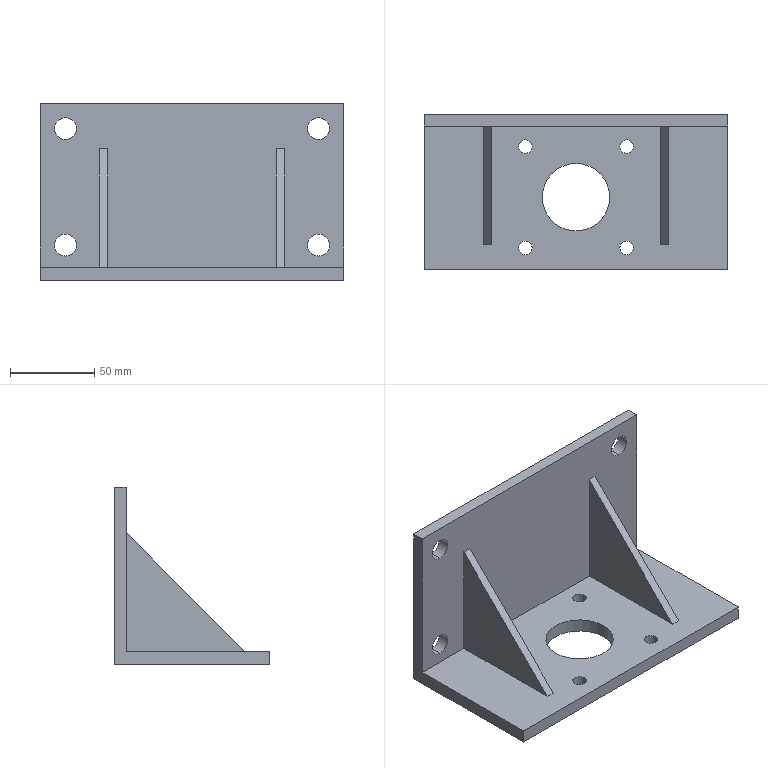Component | SolidWorks | NewTypeCurveBenderDoubleTelescopicCylinderBasePlate-DoubleWheel-2 | 1 solid | 32 faces | box 180 x 92 x 105 mm | volume 263822 mm3 | cylinder 18 | plane 14 | commonest cylinder face diameters 13 x8 8 x8 40 x2
STEP:
#1=COLOUR_RGB('',0.7922,0.8196,0.9333);
#2=FILL_AREA_STYLE_COLOUR('',#1);
#3=FILL_AREA_STYLE('',(#2));
#4=SURFACE_STYLE_FILL_AREA(#3);
#5=SURFACE_SIDE_STYLE('',(#4));
#6=SURFACE_STYLE_USAGE(.BOTH.,#5);
#7=PRESENTATION_STYLE_ASSIGNMENT((#6));
#8=CARTESIAN_POINT('',(2.953,3.504,14.04));
#9=VERTEX_POINT('',#8);
#10=CARTESIAN_POINT('',(2.953,3.504,14.552));
#11=VERTEX_POINT('',#10);
#12=CARTESIAN_POINT('',(2.953,3.504,14.296));
#13=DIRECTION('',(-0.,1.,0.));
#14=DIRECTION('',(0.,0.,1.));
#15=AXIS2_PLACEMENT_3D('',#12,#13,#14);
#16=CIRCLE('',#15,0.2559);
#17=EDGE_CURVE('',#9,#11,#16,.T.);
#18=ORIENTED_EDGE('',*,*,#17,.F.);
#19=CARTESIAN_POINT('',(2.953,3.78,14.04));
#20=VERTEX_POINT('',#19);
#21=CARTESIAN_POINT('',(2.953,3.78,14.04));
#22=DIRECTION('',(-0.,1.,0.));
#23=VECTOR('',#22,39.37);
#24=LINE('',#21,#23);
#25=EDGE_CURVE('',#9,#20,#24,.T.);
#26=ORIENTED_EDGE('',*,*,#25,.T.);
#27=CARTESIAN_POINT('',(2.953,3.78,14.552));
#28=VERTEX_POINT('',#27);
#29=CARTESIAN_POINT('',(2.953,3.78,14.296));
#30=DIRECTION('',(-0.,1.,0.));
#31=DIRECTION('',(0.,0.,1.));
#32=AXIS2_PLACEMENT_3D('',#29,#30,#31);
#33=CIRCLE('',#32,0.2559);
#34=EDGE_CURVE('',#20,#28,#33,.T.);
#35=ORIENTED_EDGE('',*,*,#34,.T.);
#36=CARTESIAN_POINT('',(2.953,3.78,14.552));
#37=DIRECTION('',(-0.,1.,0.));
#38=VECTOR('',#37,39.37);
#39=LINE('',#36,#38);
#40=EDGE_CURVE('',#11,#28,#39,.T.);
#41=ORIENTED_EDGE('',*,*,#40,.F.);
#42=EDGE_LOOP('',(#18,#26,#35,#41));
#43=FACE_OUTER_BOUND('',#42,.T.);
#44=CARTESIAN_POINT('',(2.953,3.78,14.296));
#45=DIRECTION('',(-0.,1.,0.));
#46=DIRECTION('',(0.,0.,1.));
#47=AXIS2_PLACEMENT_3D('',#44,#45,#46);
#48=CYLINDRICAL_SURFACE('',#47,0.2559);
#49=ADVANCED_FACE('',(#43),#48,.F.);
#50=CARTESIAN_POINT('',(2.953,3.504,11.323));
#51=VERTEX_POINT('',#50);
#52=CARTESIAN_POINT('',(2.953,3.504,11.835));
#53=VERTEX_POINT('',#52);
#54=CARTESIAN_POINT('',(2.953,3.504,11.579));
#55=DIRECTION('',(-0.,1.,0.));
#56=DIRECTION('',(0.,0.,1.));
#57=AXIS2_PLACEMENT_3D('',#54,#55,#56);
#58=CIRCLE('',#57,0.2559);
#59=EDGE_CURVE('',#51,#53,#58,.T.);
#60=ORIENTED_EDGE('',*,*,#59,.F.);
#61=CARTESIAN_POINT('',(2.953,3.78,11.323));
#62=VERTEX_POINT('',#61);
#63=CARTESIAN_POINT('',(2.953,3.78,11.323));
#64=DIRECTION('',(-0.,1.,0.));
#65=VECTOR('',#64,39.37);
#66=LINE('',#63,#65);
#67=EDGE_CURVE('',#51,#62,#66,.T.);
#68=ORIENTED_EDGE('',*,*,#67,.T.);
#69=CARTESIAN_POINT('',(2.953,3.78,11.835));
#70=VERTEX_POINT('',#69);
#71=CARTESIAN_POINT('',(2.953,3.78,11.579));
#72=DIRECTION('',(-0.,1.,0.));
#73=DIRECTION('',(0.,0.,1.));
#74=AXIS2_PLACEMENT_3D('',#71,#72,#73);
#75=CIRCLE('',#74,0.2559);
#76=EDGE_CURVE('',#62,#70,#75,.T.);
#77=ORIENTED_EDGE('',*,*,#76,.T.);
#78=CARTESIAN_POINT('',(2.953,3.78,11.835));
#79=DIRECTION('',(-0.,1.,0.));
#80=VECTOR('',#79,39.37);
#81=LINE('',#78,#80);
#82=EDGE_CURVE('',#53,#70,#81,.T.);
#83=ORIENTED_EDGE('',*,*,#82,.F.);
#84=EDGE_LOOP('',(#60,#68,#77,#83));
#85=FACE_OUTER_BOUND('',#84,.T.);
#86=CARTESIAN_POINT('',(2.953,3.78,11.579));
#87=DIRECTION('',(-0.,1.,0.));
#88=DIRECTION('',(0.,0.,1.));
#89=AXIS2_PLACEMENT_3D('',#86,#87,#88);
#90=CYLINDRICAL_SURFACE('',#89,0.2559);
#91=ADVANCED_FACE('',(#85),#90,.F.);
#92=CARTESIAN_POINT('',(-2.953,3.504,11.323));
#93=VERTEX_POINT('',#92);
#94=CARTESIAN_POINT('',(-2.953,3.504,11.835));
#95=VERTEX_POINT('',#94);
#96=CARTESIAN_POINT('',(-2.953,3.504,11.579));
#97=DIRECTION('',(-0.,1.,0.));
#98=DIRECTION('',(0.,0.,1.));
#99=AXIS2_PLACEMENT_3D('',#96,#97,#98);
#100=CIRCLE('',#99,0.2559);
#101=EDGE_CURVE('',#93,#95,#100,.T.);
#102=ORIENTED_EDGE('',*,*,#101,.F.);
#103=CARTESIAN_POINT('',(-2.953,3.78,11.323));
#104=VERTEX_POINT('',#103);
#105=CARTESIAN_POINT('',(-2.953,3.78,11.323));
#106=DIRECTION('',(-0.,1.,0.));
#107=VECTOR('',#106,39.37);
#108=LINE('',#105,#107);
#109=EDGE_CURVE('',#93,#104,#108,.T.);
#110=ORIENTED_EDGE('',*,*,#109,.T.);
#111=CARTESIAN_POINT('',(-2.953,3.78,11.835));
#112=VERTEX_POINT('',#111);
#113=CARTESIAN_POINT('',(-2.953,3.78,11.579));
#114=DIRECTION('',(-0.,1.,0.));
#115=DIRECTION('',(0.,0.,1.));
#116=AXIS2_PLACEMENT_3D('',#113,#114,#115);
#117=CIRCLE('',#116,0.2559);
#118=EDGE_CURVE('',#104,#112,#117,.T.);
#119=ORIENTED_EDGE('',*,*,#118,.T.);
#120=CARTESIAN_POINT('',(-2.953,3.78,11.835));
#121=DIRECTION('',(-0.,1.,0.));
#122=VECTOR('',#121,39.37);
#123=LINE('',#120,#122);
#124=EDGE_CURVE('',#95,#112,#123,.T.);
#125=ORIENTED_EDGE('',*,*,#124,.F.);
#126=EDGE_LOOP('',(#102,#110,#119,#125));
#127=FACE_OUTER_BOUND('',#126,.T.);
#128=CARTESIAN_POINT('',(-2.953,3.78,11.579));
#129=DIRECTION('',(-0.,1.,0.));
#130=DIRECTION('',(0.,0.,1.));
#131=AXIS2_PLACEMENT_3D('',#128,#129,#130);
#132=CYLINDRICAL_SURFACE('',#131,0.2559);
#133=ADVANCED_FACE('',(#127),#132,.F.);
#134=CARTESIAN_POINT('',(-2.953,3.504,14.04));
#135=VERTEX_POINT('',#134);
#136=CARTESIAN_POINT('',(-2.953,3.504,14.552));
#137=VERTEX_POINT('',#136);
#138=CARTESIAN_POINT('',(-2.953,3.504,14.296));
#139=DIRECTION('',(-0.,1.,0.));
#140=DIRECTION('',(0.,0.,1.));
#141=AXIS2_PLACEMENT_3D('',#138,#139,#140);
#142=CIRCLE('',#141,0.2559);
#143=EDGE_CURVE('',#135,#137,#142,.T.);
#144=ORIENTED_EDGE('',*,*,#143,.F.);
#145=CARTESIAN_POINT('',(-2.953,3.78,14.04));
#146=VERTEX_POINT('',#145);
#147=CARTESIAN_POINT('',(-2.953,3.78,14.04));
#148=DIRECTION('',(-0.,1.,0.));
#149=VECTOR('',#148,39.37);
#150=LINE('',#147,#149);
#151=EDGE_CURVE('',#135,#146,#150,.T.);
#152=ORIENTED_EDGE('',*,*,#151,.T.);
#153=CARTESIAN_POINT('',(-2.953,3.78,14.552));
#154=VERTEX_POINT('',#153);
#155=CARTESIAN_POINT('',(-2.953,3.78,14.296));
#156=DIRECTION('',(-0.,1.,0.));
#157=DIRECTION('',(0.,0.,1.));
#158=AXIS2_PLACEMENT_3D('',#155,#156,#157);
#159=CIRCLE('',#158,0.2559);
#160=EDGE_CURVE('',#146,#154,#159,.T.);
#161=ORIENTED_EDGE('',*,*,#160,.T.);
#162=CARTESIAN_POINT('',(-2.953,3.78,14.552));
#163=DIRECTION('',(-0.,1.,0.));
#164=VECTOR('',#163,39.37);
#165=LINE('',#162,#164);
#166=EDGE_CURVE('',#137,#154,#165,.T.);
#167=ORIENTED_EDGE('',*,*,#166,.F.);
#168=EDGE_LOOP('',(#144,#152,#161,#167));
#169=FACE_OUTER_BOUND('',#168,.T.);
#170=CARTESIAN_POINT('',(-2.953,3.78,14.296));
#171=DIRECTION('',(-0.,1.,0.));
#172=DIRECTION('',(0.,0.,1.));
#173=AXIS2_PLACEMENT_3D('',#170,#171,#172);
#174=CYLINDRICAL_SURFACE('',#173,0.2559);
#175=ADVANCED_FACE('',(#169),#174,.F.);
#176=CARTESIAN_POINT('',(-1.339,3.031,11.067));
#177=VERTEX_POINT('',#176);
#178=CARTESIAN_POINT('',(-1.024,3.031,11.067));
#179=VERTEX_POINT('',#178);
#180=CARTESIAN_POINT('',(-1.181,3.031,11.067));
#181=DIRECTION('',(-0.,0.,-1.));
#182=DIRECTION('',(1.,0.,0.));
#183=AXIS2_PLACEMENT_3D('',#180,#181,#182);
#184=CIRCLE('',#183,0.1575);
#185=EDGE_CURVE('',#177,#179,#184,.T.);
#186=ORIENTED_EDGE('',*,*,#185,.F.);
#187=CARTESIAN_POINT('',(-1.339,3.031,10.752));
#188=VERTEX_POINT('',#187);
#189=CARTESIAN_POINT('',(-1.339,3.031,11.146));
#190=DIRECTION('',(-0.,0.,-1.));
#191=VECTOR('',#190,39.37);
#192=LINE('',#189,#191);
#193=EDGE_CURVE('',#177,#188,#192,.T.);
#194=ORIENTED_EDGE('',*,*,#193,.T.);
#195=CARTESIAN_POINT('',(-1.024,3.031,10.752));
#196=VERTEX_POINT('',#195);
#197=CARTESIAN_POINT('',(-1.181,3.031,10.752));
#198=DIRECTION('',(-0.,0.,-1.));
#199=DIRECTION('',(-1.,0.,0.));
#200=AXIS2_PLACEMENT_3D('',#197,#198,#199);
#201=CIRCLE('',#200,0.1575);
#202=EDGE_CURVE('',#188,#196,#201,.T.);
#203=ORIENTED_EDGE('',*,*,#202,.T.);
#204=CARTESIAN_POINT('',(-1.024,3.031,11.146));
#205=DIRECTION('',(-0.,0.,-1.));
#206=VECTOR('',#205,39.37);
#207=LINE('',#204,#206);
#208=EDGE_CURVE('',#179,#196,#207,.T.);
#209=ORIENTED_EDGE('',*,*,#208,.F.);
#210=EDGE_LOOP('',(#186,#194,#203,#209));
#211=FACE_OUTER_BOUND('',#210,.T.);
#212=CARTESIAN_POINT('',(-1.181,3.031,11.146));
#213=DIRECTION('',(-0.,0.,-1.));
#214=DIRECTION('',(1.,0.,0.));
#215=AXIS2_PLACEMENT_3D('',#212,#213,#214);
#216=CYLINDRICAL_SURFACE('',#215,0.1575);
#217=ADVANCED_FACE('',(#211),#216,.F.);
#218=CARTESIAN_POINT('',(1.024,3.031,11.067));
#219=VERTEX_POINT('',#218);
#220=CARTESIAN_POINT('',(1.339,3.031,11.067));
#221=VERTEX_POINT('',#220);
#222=CARTESIAN_POINT('',(1.181,3.031,11.067));
#223=DIRECTION('',(-0.,0.,-1.));
#224=DIRECTION('',(1.,0.,0.));
#225=AXIS2_PLACEMENT_3D('',#222,#223,#224);
#226=CIRCLE('',#225,0.1575);
#227=EDGE_CURVE('',#219,#221,#226,.T.);
#228=ORIENTED_EDGE('',*,*,#227,.F.);
#229=CARTESIAN_POINT('',(1.024,3.031,10.752));
#230=VERTEX_POINT('',#229);
#231=CARTESIAN_POINT('',(1.024,3.031,11.146));
#232=DIRECTION('',(-0.,0.,-1.));
#233=VECTOR('',#232,39.37);
#234=LINE('',#231,#233);
#235=EDGE_CURVE('',#219,#230,#234,.T.);
#236=ORIENTED_EDGE('',*,*,#235,.T.);
#237=CARTESIAN_POINT('',(1.339,3.031,10.752));
#238=VERTEX_POINT('',#237);
#239=CARTESIAN_POINT('',(1.181,3.031,10.752));
#240=DIRECTION('',(-0.,0.,-1.));
#241=DIRECTION('',(1.,0.,0.));
#242=AXIS2_PLACEMENT_3D('',#239,#240,#241);
#243=CIRCLE('',#242,0.1575);
#244=EDGE_CURVE('',#230,#238,#243,.T.);
#245=ORIENTED_EDGE('',*,*,#244,.T.);
#246=CARTESIAN_POINT('',(1.339,3.031,11.146));
#247=DIRECTION('',(-0.,0.,-1.));
#248=VECTOR('',#247,39.37);
#249=LINE('',#246,#248);
#250=EDGE_CURVE('',#221,#238,#249,.T.);
#251=ORIENTED_EDGE('',*,*,#250,.F.);
#252=EDGE_LOOP('',(#228,#236,#245,#251));
#253=FACE_OUTER_BOUND('',#252,.T.);
#254=CARTESIAN_POINT('',(1.181,3.031,11.146));
#255=DIRECTION('',(-0.,0.,-1.));
#256=DIRECTION('',(1.,0.,0.));
#257=AXIS2_PLACEMENT_3D('',#254,#255,#256);
#258=CYLINDRICAL_SURFACE('',#257,0.1575);
#259=ADVANCED_FACE('',(#253),#258,.F.);
#260=CARTESIAN_POINT('',(1.024,0.6693,11.067));
#261=VERTEX_POINT('',#260);
#262=CARTESIAN_POINT('',(1.339,0.6693,11.067));
#263=VERTEX_POINT('',#262);
#264=CARTESIAN_POINT('',(1.181,0.6693,11.067));
#265=DIRECTION('',(-0.,0.,-1.));
#266=DIRECTION('',(1.,0.,0.));
#267=AXIS2_PLACEMENT_3D('',#264,#265,#266);
#268=CIRCLE('',#267,0.1575);
#269=EDGE_CURVE('',#261,#263,#268,.T.);
#270=ORIENTED_EDGE('',*,*,#269,.F.);
#271=CARTESIAN_POINT('',(1.024,0.6693,10.752));
#272=VERTEX_POINT('',#271);
#273=CARTESIAN_POINT('',(1.024,0.6693,11.146));
#274=DIRECTION('',(-0.,0.,-1.));
#275=VECTOR('',#274,39.37);
#276=LINE('',#273,#275);
#277=EDGE_CURVE('',#261,#272,#276,.T.);
#278=ORIENTED_EDGE('',*,*,#277,.T.);
#279=CARTESIAN_POINT('',(1.339,0.6693,10.752));
#280=VERTEX_POINT('',#279);
#281=CARTESIAN_POINT('',(1.181,0.6693,10.752));
#282=DIRECTION('',(-0.,0.,-1.));
#283=DIRECTION('',(-1.,0.,0.));
#284=AXIS2_PLACEMENT_3D('',#281,#282,#283);
#285=CIRCLE('',#284,0.1575);
#286=EDGE_CURVE('',#272,#280,#285,.T.);
#287=ORIENTED_EDGE('',*,*,#286,.T.);
#288=CARTESIAN_POINT('',(1.339,0.6693,11.146));
#289=DIRECTION('',(-0.,0.,-1.));
#290=VECTOR('',#289,39.37);
#291=LINE('',#288,#290);
#292=EDGE_CURVE('',#263,#280,#291,.T.);
#293=ORIENTED_EDGE('',*,*,#292,.F.);
#294=EDGE_LOOP('',(#270,#278,#287,#293));
#295=FACE_OUTER_BOUND('',#294,.T.);
#296=CARTESIAN_POINT('',(1.181,0.6693,11.146));
#297=DIRECTION('',(-0.,0.,-1.));
#298=DIRECTION('',(1.,0.,0.));
#299=AXIS2_PLACEMENT_3D('',#296,#297,#298);
#300=CYLINDRICAL_SURFACE('',#299,0.1575);
#301=ADVANCED_FACE('',(#295),#300,.F.);
#302=CARTESIAN_POINT('',(-1.339,0.6693,11.067));
#303=VERTEX_POINT('',#302);
#304=CARTESIAN_POINT('',(-1.024,0.6693,11.067));
#305=VERTEX_POINT('',#304);
#306=CARTESIAN_POINT('',(-1.181,0.6693,11.067));
#307=DIRECTION('',(-0.,0.,-1.));
#308=DIRECTION('',(1.,0.,0.));
#309=AXIS2_PLACEMENT_3D('',#306,#307,#308);
#310=CIRCLE('',#309,0.1575);
#311=EDGE_CURVE('',#303,#305,#310,.T.);
#312=ORIENTED_EDGE('',*,*,#311,.F.);
#313=CARTESIAN_POINT('',(-1.339,0.6693,10.752));
#314=VERTEX_POINT('',#313);
#315=CARTESIAN_POINT('',(-1.339,0.6693,11.146));
#316=DIRECTION('',(-0.,0.,-1.));
#317=VECTOR('',#316,39.37);
#318=LINE('',#315,#317);
#319=EDGE_CURVE('',#303,#314,#318,.T.);
#320=ORIENTED_EDGE('',*,*,#319,.T.);
#321=CARTESIAN_POINT('',(-1.024,0.6693,10.752));
#322=VERTEX_POINT('',#321);
#323=CARTESIAN_POINT('',(-1.181,0.6693,10.752));
#324=DIRECTION('',(-0.,0.,-1.));
#325=DIRECTION('',(1.,0.,0.));
#326=AXIS2_PLACEMENT_3D('',#323,#324,#325);
#327=CIRCLE('',#326,0.1575);
#328=EDGE_CURVE('',#314,#322,#327,.T.);
#329=ORIENTED_EDGE('',*,*,#328,.T.);
#330=CARTESIAN_POINT('',(-1.024,0.6693,11.146));
#331=DIRECTION('',(-0.,0.,-1.));
#332=VECTOR('',#331,39.37);
#333=LINE('',#330,#332);
#334=EDGE_CURVE('',#305,#322,#333,.T.);
#335=ORIENTED_EDGE('',*,*,#334,.F.);
#336=EDGE_LOOP('',(#312,#320,#329,#335));
#337=FACE_OUTER_BOUND('',#336,.T.);
#338=CARTESIAN_POINT('',(-1.181,0.6693,11.146));
#339=DIRECTION('',(-0.,0.,-1.));
#340=DIRECTION('',(1.,0.,0.));
#341=AXIS2_PLACEMENT_3D('',#338,#339,#340);
#342=CYLINDRICAL_SURFACE('',#341,0.1575);
#343=ADVANCED_FACE('',(#337),#342,.F.);
#344=CARTESIAN_POINT('',(-0.7874,1.85,11.067));
#345=VERTEX_POINT('',#344);
#346=CARTESIAN_POINT('',(0.7874,1.85,11.067));
#347=VERTEX_POINT('',#346);
#348=CARTESIAN_POINT('',(-0.,1.85,11.067));
#349=DIRECTION('',(-0.,0.,-1.));
#350=DIRECTION('',(1.,0.,0.));
#351=AXIS2_PLACEMENT_3D('',#348,#349,#350);
#352=CIRCLE('',#351,0.7874);
#353=EDGE_CURVE('',#345,#347,#352,.T.);
#354=ORIENTED_EDGE('',*,*,#353,.F.);
#355=CARTESIAN_POINT('',(-0.7874,1.85,10.752));
#356=VERTEX_POINT('',#355);
#357=CARTESIAN_POINT('',(-0.7874,1.85,11.146));
#358=DIRECTION('',(-0.,0.,-1.));
#359=VECTOR('',#358,39.37);
#360=LINE('',#357,#359);
#361=EDGE_CURVE('',#345,#356,#360,.T.);
#362=ORIENTED_EDGE('',*,*,#361,.T.);
#363=CARTESIAN_POINT('',(0.7874,1.85,10.752));
#364=VERTEX_POINT('',#363);
#365=CARTESIAN_POINT('',(-0.,1.85,10.752));
#366=DIRECTION('',(-0.,0.,-1.));
#367=DIRECTION('',(1.,0.,0.));
#368=AXIS2_PLACEMENT_3D('',#365,#366,#367);
#369=CIRCLE('',#368,0.7874);
#370=EDGE_CURVE('',#356,#364,#369,.T.);
#371=ORIENTED_EDGE('',*,*,#370,.T.);
#372=CARTESIAN_POINT('',(0.7874,1.85,11.146));
#373=DIRECTION('',(-0.,0.,-1.));
#374=VECTOR('',#373,39.37);
#375=LINE('',#372,#374);
#376=EDGE_CURVE('',#347,#364,#375,.T.);
#377=ORIENTED_EDGE('',*,*,#376,.F.);
#378=EDGE_LOOP('',(#354,#362,#371,#377));
#379=FACE_OUTER_BOUND('',#378,.T.);
#380=CARTESIAN_POINT('',(-0.,1.85,11.146));
#381=DIRECTION('',(-0.,0.,-1.));
#382=DIRECTION('',(1.,0.,0.));
#383=AXIS2_PLACEMENT_3D('',#380,#381,#382);
#384=CYLINDRICAL_SURFACE('',#383,0.7874);
#385=ADVANCED_FACE('',(#379),#384,.F.);
#386=CARTESIAN_POINT('',(-0.,1.85,11.067));
#387=DIRECTION('',(-0.,0.,-1.));
#388=DIRECTION('',(1.,0.,0.));
#389=AXIS2_PLACEMENT_3D('',#386,#387,#388);
#390=CIRCLE('',#389,0.7874);
#391=EDGE_CURVE('',#347,#345,#390,.T.);
#392=ORIENTED_EDGE('',*,*,#391,.T.);
#393=ORIENTED_EDGE('',*,*,#353,.T.);
#394=EDGE_LOOP('',(#392,#393));
#395=FACE_BOUND('',#394,.T.);
#396=CARTESIAN_POINT('',(-1.181,0.6693,11.067));
#397=DIRECTION('',(-0.,0.,-1.));
#398=DIRECTION('',(1.,0.,0.));
#399=AXIS2_PLACEMENT_3D('',#396,#397,#398);
#400=CIRCLE('',#399,0.1575);
#401=EDGE_CURVE('',#305,#303,#400,.T.);
#402=ORIENTED_EDGE('',*,*,#401,.T.);
#403=ORIENTED_EDGE('',*,*,#311,.T.);
#404=EDGE_LOOP('',(#402,#403));
#405=FACE_BOUND('',#404,.T.);
#406=CARTESIAN_POINT('',(1.181,0.6693,11.067));
#407=DIRECTION('',(-0.,0.,-1.));
#408=DIRECTION('',(1.,0.,0.));
#409=AXIS2_PLACEMENT_3D('',#406,#407,#408);
#410=CIRCLE('',#409,0.1575);
#411=EDGE_CURVE('',#263,#261,#410,.T.);
#412=ORIENTED_EDGE('',*,*,#411,.T.);
#413=ORIENTED_EDGE('',*,*,#269,.T.);
#414=EDGE_LOOP('',(#412,#413));
#415=FACE_BOUND('',#414,.T.);
#416=CARTESIAN_POINT('',(1.181,3.031,11.067));
#417=DIRECTION('',(-0.,0.,-1.));
#418=DIRECTION('',(1.,0.,0.));
#419=AXIS2_PLACEMENT_3D('',#416,#417,#418);
#420=CIRCLE('',#419,0.1575);
#421=EDGE_CURVE('',#221,#219,#420,.T.);
#422=ORIENTED_EDGE('',*,*,#421,.T.);
#423=ORIENTED_EDGE('',*,*,#227,.T.);
#424=EDGE_LOOP('',(#422,#423));
#425=FACE_BOUND('',#424,.T.);
#426=CARTESIAN_POINT('',(-1.181,3.031,11.067));
#427=DIRECTION('',(-0.,0.,-1.));
#428=DIRECTION('',(1.,0.,0.));
#429=AXIS2_PLACEMENT_3D('',#426,#427,#428);
#430=CIRCLE('',#429,0.1575);
#431=EDGE_CURVE('',#179,#177,#430,.T.);
#432=ORIENTED_EDGE('',*,*,#431,.T.);
#433=ORIENTED_EDGE('',*,*,#185,.T.);
#434=EDGE_LOOP('',(#432,#433));
#435=FACE_BOUND('',#434,.T.);
#436=CARTESIAN_POINT('',(1.969,0.748,11.067));
#437=VERTEX_POINT('',#436);
#438=CARTESIAN_POINT('',(2.165,0.748,11.067));
#439=VERTEX_POINT('',#438);
#440=CARTESIAN_POINT('',(1.969,0.748,11.067));
#441=DIRECTION('',(1.,0.,-0.));
#442=VECTOR('',#441,39.37);
#443=LINE('',#440,#442);
#444=EDGE_CURVE('',#437,#439,#443,.T.);
#445=ORIENTED_EDGE('',*,*,#444,.F.);
#446=CARTESIAN_POINT('',(1.969,3.504,11.067));
#447=VERTEX_POINT('',#446);
#448=CARTESIAN_POINT('',(1.969,3.504,11.067));
#449=DIRECTION('',(0.,-1.,-0.));
#450=VECTOR('',#449,39.37);
#451=LINE('',#448,#450);
#452=EDGE_CURVE('',#447,#437,#451,.T.);
#453=ORIENTED_EDGE('',*,*,#452,.F.);
#454=CARTESIAN_POINT('',(-1.969,3.504,11.067));
#455=VERTEX_POINT('',#454);
#456=CARTESIAN_POINT('',(3.543,3.504,11.067));
#457=DIRECTION('',(1.,0.,-0.));
#458=VECTOR('',#457,39.37);
#459=LINE('',#456,#458);
#460=EDGE_CURVE('',#455,#447,#459,.T.);
#461=ORIENTED_EDGE('',*,*,#460,.F.);
#462=CARTESIAN_POINT('',(-1.969,0.748,11.067));
#463=VERTEX_POINT('',#462);
#464=CARTESIAN_POINT('',(-1.969,3.504,11.067));
#465=DIRECTION('',(-0.,-1.,-0.));
#466=VECTOR('',#465,39.37);
#467=LINE('',#464,#466);
#468=EDGE_CURVE('',#455,#463,#467,.T.);
#469=ORIENTED_EDGE('',*,*,#468,.T.);
#470=CARTESIAN_POINT('',(-2.165,0.748,11.067));
#471=VERTEX_POINT('',#470);
#472=CARTESIAN_POINT('',(-1.969,0.748,11.067));
#473=DIRECTION('',(-1.,0.,0.));
#474=VECTOR('',#473,39.37);
#475=LINE('',#472,#474);
#476=EDGE_CURVE('',#463,#471,#475,.T.);
#477=ORIENTED_EDGE('',*,*,#476,.T.);
#478=CARTESIAN_POINT('',(-2.165,3.504,11.067));
#479=VERTEX_POINT('',#478);
#480=CARTESIAN_POINT('',(-2.165,3.504,11.067));
#481=DIRECTION('',(-0.,-1.,-0.));
#482=VECTOR('',#481,39.37);
#483=LINE('',#480,#482);
#484=EDGE_CURVE('',#479,#471,#483,.T.);
#485=ORIENTED_EDGE('',*,*,#484,.F.);
#486=CARTESIAN_POINT('',(-3.543,3.504,11.067));
#487=VERTEX_POINT('',#486);
#488=CARTESIAN_POINT('',(3.543,3.504,11.067));
#489=DIRECTION('',(1.,0.,-0.));
#490=VECTOR('',#489,39.37);
#491=LINE('',#488,#490);
#492=EDGE_CURVE('',#487,#479,#491,.T.);
#493=ORIENTED_EDGE('',*,*,#492,.F.);
#494=CARTESIAN_POINT('',(-3.543,0.1575,11.067));
#495=VERTEX_POINT('',#494);
#496=CARTESIAN_POINT('',(-3.543,0.1575,11.067));
#497=DIRECTION('',(-0.,1.,0.));
#498=VECTOR('',#497,39.37);
#499=LINE('',#496,#498);
#500=EDGE_CURVE('',#495,#487,#499,.T.);
#501=ORIENTED_EDGE('',*,*,#500,.F.);
#502=CARTESIAN_POINT('',(3.543,0.1575,11.067));
#503=VERTEX_POINT('',#502);
#504=CARTESIAN_POINT('',(-3.543,0.1575,11.067));
#505=DIRECTION('',(-1.,-0.,0.));
#506=VECTOR('',#505,39.37);
#507=LINE('',#504,#506);
#508=EDGE_CURVE('',#503,#495,#507,.T.);
#509=ORIENTED_EDGE('',*,*,#508,.F.);
#510=CARTESIAN_POINT('',(3.543,3.504,11.067));
#511=VERTEX_POINT('',#510);
#512=CARTESIAN_POINT('',(3.543,0.1575,11.067));
#513=DIRECTION('',(0.,-1.,-0.));
#514=VECTOR('',#513,39.37);
#515=LINE('',#512,#514);
#516=EDGE_CURVE('',#511,#503,#515,.T.);
#517=ORIENTED_EDGE('',*,*,#516,.F.);
#518=CARTESIAN_POINT('',(2.165,3.504,11.067));
#519=VERTEX_POINT('',#518);
#520=CARTESIAN_POINT('',(3.543,3.504,11.067));
#521=DIRECTION('',(1.,0.,-0.));
#522=VECTOR('',#521,39.37);
#523=LINE('',#520,#522);
#524=EDGE_CURVE('',#519,#511,#523,.T.);
#525=ORIENTED_EDGE('',*,*,#524,.F.);
#526=CARTESIAN_POINT('',(2.165,3.504,11.067));
#527=DIRECTION('',(0.,-1.,-0.));
#528=VECTOR('',#527,39.37);
#529=LINE('',#526,#528);
#530=EDGE_CURVE('',#519,#439,#529,.T.);
#531=ORIENTED_EDGE('',*,*,#530,.T.);
#532=EDGE_LOOP('',(#445,#453,#461,#469,#477,#485,#493,#501,#509,#517,#525,#531));
#533=FACE_OUTER_BOUND('',#532,.T.);
#534=CARTESIAN_POINT('',(-0.,1.988,11.067));
#535=DIRECTION('',(-0.,0.,-1.));
#536=DIRECTION('',(1.,0.,-0.));
#537=AXIS2_PLACEMENT_3D('',#534,#535,#536);
#538=PLANE('',#537);
#539=ADVANCED_FACE('',(#395,#405,#415,#425,#435,#533),#538,.F.);
#540=CARTESIAN_POINT('',(3.543,3.78,10.752));
#541=VERTEX_POINT('',#540);
#542=CARTESIAN_POINT('',(3.543,0.1575,10.752));
#543=VERTEX_POINT('',#542);
#544=CARTESIAN_POINT('',(3.543,0.1575,10.752));
#545=DIRECTION('',(0.,-1.,-0.));
#546=VECTOR('',#545,39.37);
#547=LINE('',#544,#546);
#548=EDGE_CURVE('',#541,#543,#547,.T.);
#549=ORIENTED_EDGE('',*,*,#548,.F.);
#550=CARTESIAN_POINT('',(3.543,3.78,14.886));
#551=VERTEX_POINT('',#550);
#552=CARTESIAN_POINT('',(3.543,3.78,14.886));
#553=DIRECTION('',(-0.,0.,-1.));
#554=VECTOR('',#553,39.37);
#555=LINE('',#552,#554);
#556=EDGE_CURVE('',#551,#541,#555,.T.);
#557=ORIENTED_EDGE('',*,*,#556,.F.);
#558=CARTESIAN_POINT('',(3.543,3.504,14.886));
#559=VERTEX_POINT('',#558);
#560=CARTESIAN_POINT('',(3.543,3.78,14.886));
#561=DIRECTION('',(-0.,1.,0.));
#562=VECTOR('',#561,39.37);
#563=LINE('',#560,#562);
#564=EDGE_CURVE('',#559,#551,#563,.T.);
#565=ORIENTED_EDGE('',*,*,#564,.F.);
#566=CARTESIAN_POINT('',(3.543,3.504,14.886));
#567=DIRECTION('',(-0.,0.,-1.));
#568=VECTOR('',#567,39.37);
#569=LINE('',#566,#568);
#570=EDGE_CURVE('',#559,#511,#569,.T.);
#571=ORIENTED_EDGE('',*,*,#570,.T.);
#572=ORIENTED_EDGE('',*,*,#516,.T.);
#573=CARTESIAN_POINT('',(3.543,0.1575,10.752));
#574=DIRECTION('',(0.,-0.,1.));
#575=VECTOR('',#574,39.37);
#576=LINE('',#573,#575);
#577=EDGE_CURVE('',#543,#503,#576,.T.);
#578=ORIENTED_EDGE('',*,*,#577,.F.);
#579=EDGE_LOOP('',(#549,#557,#565,#571,#572,#578));
#580=FACE_OUTER_BOUND('',#579,.T.);
#581=CARTESIAN_POINT('',(3.543,0.1575,10.752));
#582=DIRECTION('',(-1.,-0.,0.));
#583=DIRECTION('',(-0.,0.,-1.));
#584=AXIS2_PLACEMENT_3D('',#581,#582,#583);
#585=PLANE('',#584);
#586=ADVANCED_FACE('',(#580),#585,.F.);
#587=ORIENTED_EDGE('',*,*,#508,.T.);
#588=CARTESIAN_POINT('',(-3.543,0.1575,10.752));
#589=VERTEX_POINT('',#588);
#590=CARTESIAN_POINT('',(-3.543,0.1575,10.752));
#591=DIRECTION('',(0.,-0.,1.));
#592=VECTOR('',#591,39.37);
#593=LINE('',#590,#592);
#594=EDGE_CURVE('',#589,#495,#593,.T.);
#595=ORIENTED_EDGE('',*,*,#594,.F.);
#596=CARTESIAN_POINT('',(-3.543,0.1575,10.752));
#597=DIRECTION('',(-1.,-0.,0.));
#598=VECTOR('',#597,39.37);
#599=LINE('',#596,#598);
#600=EDGE_CURVE('',#543,#589,#599,.T.);
#601=ORIENTED_EDGE('',*,*,#600,.F.);
#602=ORIENTED_EDGE('',*,*,#577,.T.);
#603=EDGE_LOOP('',(#587,#595,#601,#602));
#604=FACE_OUTER_BOUND('',#603,.T.);
#605=CARTESIAN_POINT('',(-3.543,0.1575,10.752));
#606=DIRECTION('',(-0.,1.,0.));
#607=DIRECTION('',(0.,-0.,1.));
#608=AXIS2_PLACEMENT_3D('',#605,#606,#607);
#609=PLANE('',#608);
#610=ADVANCED_FACE('',(#604),#609,.F.);
#611=CARTESIAN_POINT('',(-3.543,3.78,14.886));
#612=VERTEX_POINT('',#611);
#613=CARTESIAN_POINT('',(-3.543,3.78,10.752));
#614=VERTEX_POINT('',#613);
#615=CARTESIAN_POINT('',(-3.543,3.78,14.886));
#616=DIRECTION('',(-0.,0.,-1.));
#617=VECTOR('',#616,39.37);
#618=LINE('',#615,#617);
#619=EDGE_CURVE('',#612,#614,#618,.T.);
#620=ORIENTED_EDGE('',*,*,#619,.T.);
#621=CARTESIAN_POINT('',(-3.543,0.1575,10.752));
#622=DIRECTION('',(-0.,1.,0.));
#623=VECTOR('',#622,39.37);
#624=LINE('',#621,#623);
#625=EDGE_CURVE('',#589,#614,#624,.T.);
#626=ORIENTED_EDGE('',*,*,#625,.F.);
#627=ORIENTED_EDGE('',*,*,#594,.T.);
#628=ORIENTED_EDGE('',*,*,#500,.T.);
#629=CARTESIAN_POINT('',(-3.543,3.504,14.886));
#630=VERTEX_POINT('',#629);
#631=CARTESIAN_POINT('',(-3.543,3.504,14.886));
#632=DIRECTION('',(-0.,0.,-1.));
#633=VECTOR('',#632,39.37);
#634=LINE('',#631,#633);
#635=EDGE_CURVE('',#630,#487,#634,.T.);
#636=ORIENTED_EDGE('',*,*,#635,.F.);
#637=CARTESIAN_POINT('',(-3.543,3.78,14.886));
#638=DIRECTION('',(-0.,-1.,-0.));
#639=VECTOR('',#638,39.37);
#640=LINE('',#637,#639);
#641=EDGE_CURVE('',#612,#630,#640,.T.);
#642=ORIENTED_EDGE('',*,*,#641,.F.);
#643=EDGE_LOOP('',(#620,#626,#627,#628,#636,#642));
#644=FACE_OUTER_BOUND('',#643,.T.);
#645=CARTESIAN_POINT('',(-3.543,0.1575,10.752));
#646=DIRECTION('',(1.,0.,-0.));
#647=DIRECTION('',(0.,-1.,-0.));
#648=AXIS2_PLACEMENT_3D('',#645,#646,#647);
#649=PLANE('',#648);
#650=ADVANCED_FACE('',(#644),#649,.F.);
#651=CARTESIAN_POINT('',(-0.,3.78,10.752));
#652=DIRECTION('',(-1.,-0.,0.));
#653=VECTOR('',#652,39.37);
#654=LINE('',#651,#653);
#655=EDGE_CURVE('',#541,#614,#654,.T.);
#656=ORIENTED_EDGE('',*,*,#655,.F.);
#657=ORIENTED_EDGE('',*,*,#548,.T.);
#658=ORIENTED_EDGE('',*,*,#600,.T.);
#659=ORIENTED_EDGE('',*,*,#625,.T.);
#660=EDGE_LOOP('',(#656,#657,#658,#659));
#661=FACE_OUTER_BOUND('',#660,.T.);
#662=CARTESIAN_POINT('',(-1.181,3.031,10.752));
#663=DIRECTION('',(-0.,0.,-1.));
#664=DIRECTION('',(-1.,0.,0.));
#665=AXIS2_PLACEMENT_3D('',#662,#663,#664);
#666=CIRCLE('',#665,0.1575);
#667=EDGE_CURVE('',#196,#188,#666,.T.);
#668=ORIENTED_EDGE('',*,*,#667,.F.);
#669=ORIENTED_EDGE('',*,*,#202,.F.);
#670=EDGE_LOOP('',(#668,#669));
#671=FACE_BOUND('',#670,.T.);
#672=CARTESIAN_POINT('',(1.181,3.031,10.752));
#673=DIRECTION('',(-0.,0.,-1.));
#674=DIRECTION('',(1.,0.,0.));
#675=AXIS2_PLACEMENT_3D('',#672,#673,#674);
#676=CIRCLE('',#675,0.1575);
#677=EDGE_CURVE('',#238,#230,#676,.T.);
#678=ORIENTED_EDGE('',*,*,#677,.F.);
#679=ORIENTED_EDGE('',*,*,#244,.F.);
#680=EDGE_LOOP('',(#678,#679));
#681=FACE_BOUND('',#680,.T.);
#682=CARTESIAN_POINT('',(1.181,0.6693,10.752));
#683=DIRECTION('',(-0.,0.,-1.));
#684=DIRECTION('',(-1.,0.,0.));
#685=AXIS2_PLACEMENT_3D('',#682,#683,#684);
#686=CIRCLE('',#685,0.1575);
#687=EDGE_CURVE('',#280,#272,#686,.T.);
#688=ORIENTED_EDGE('',*,*,#687,.F.);
#689=ORIENTED_EDGE('',*,*,#286,.F.);
#690=EDGE_LOOP('',(#688,#689));
#691=FACE_BOUND('',#690,.T.);
#692=CARTESIAN_POINT('',(-1.181,0.6693,10.752));
#693=DIRECTION('',(-0.,0.,-1.));
#694=DIRECTION('',(1.,0.,0.));
#695=AXIS2_PLACEMENT_3D('',#692,#693,#694);
#696=CIRCLE('',#695,0.1575);
#697=EDGE_CURVE('',#322,#314,#696,.T.);
#698=ORIENTED_EDGE('',*,*,#697,.F.);
#699=ORIENTED_EDGE('',*,*,#328,.F.);
#700=EDGE_LOOP('',(#698,#699));
#701=FACE_BOUND('',#700,.T.);
#702=CARTESIAN_POINT('',(-0.,1.85,10.752));
#703=DIRECTION('',(-0.,0.,-1.));
#704=DIRECTION('',(1.,0.,0.));
#705=AXIS2_PLACEMENT_3D('',#702,#703,#704);
#706=CIRCLE('',#705,0.7874);
#707=EDGE_CURVE('',#364,#356,#706,.T.);
#708=ORIENTED_EDGE('',*,*,#707,.F.);
#709=ORIENTED_EDGE('',*,*,#370,.F.);
#710=EDGE_LOOP('',(#708,#709));
#711=FACE_BOUND('',#710,.T.);
#712=CARTESIAN_POINT('',(-0.,1.988,10.752));
#713=DIRECTION('',(-0.,0.,-1.));
#714=DIRECTION('',(1.,0.,-0.));
#715=AXIS2_PLACEMENT_3D('',#712,#713,#714);
#716=PLANE('',#715);
#717=ADVANCED_FACE('',(#661,#671,#681,#691,#701,#711),#716,.T.);
#718=ORIENTED_EDGE('',*,*,#361,.F.);
#719=ORIENTED_EDGE('',*,*,#391,.F.);
#720=ORIENTED_EDGE('',*,*,#376,.T.);
#721=ORIENTED_EDGE('',*,*,#707,.T.);
#722=EDGE_LOOP('',(#718,#719,#720,#721));
#723=FACE_OUTER_BOUND('',#722,.T.);
#724=CARTESIAN_POINT('',(-0.,1.85,11.146));
#725=DIRECTION('',(-0.,0.,-1.));
#726=DIRECTION('',(1.,0.,0.));
#727=AXIS2_PLACEMENT_3D('',#724,#725,#726);
#728=CYLINDRICAL_SURFACE('',#727,0.7874);
#729=ADVANCED_FACE('',(#723),#728,.F.);
#730=ORIENTED_EDGE('',*,*,#319,.F.);
#731=ORIENTED_EDGE('',*,*,#401,.F.);
#732=ORIENTED_EDGE('',*,*,#334,.T.);
#733=ORIENTED_EDGE('',*,*,#697,.T.);
#734=EDGE_LOOP('',(#730,#731,#732,#733));
#735=FACE_OUTER_BOUND('',#734,.T.);
#736=CARTESIAN_POINT('',(-1.181,0.6693,11.146));
#737=DIRECTION('',(-0.,0.,-1.));
#738=DIRECTION('',(1.,0.,0.));
#739=AXIS2_PLACEMENT_3D('',#736,#737,#738);
#740=CYLINDRICAL_SURFACE('',#739,0.1575);
#741=ADVANCED_FACE('',(#735),#740,.F.);
#742=ORIENTED_EDGE('',*,*,#277,.F.);
#743=ORIENTED_EDGE('',*,*,#411,.F.);
#744=ORIENTED_EDGE('',*,*,#292,.T.);
#745=ORIENTED_EDGE('',*,*,#687,.T.);
#746=EDGE_LOOP('',(#742,#743,#744,#745));
#747=FACE_OUTER_BOUND('',#746,.T.);
#748=CARTESIAN_POINT('',(1.181,0.6693,11.146));
#749=DIRECTION('',(-0.,0.,-1.));
#750=DIRECTION('',(1.,0.,0.));
#751=AXIS2_PLACEMENT_3D('',#748,#749,#750);
#752=CYLINDRICAL_SURFACE('',#751,0.1575);
#753=ADVANCED_FACE('',(#747),#752,.F.);
#754=ORIENTED_EDGE('',*,*,#235,.F.);
#755=ORIENTED_EDGE('',*,*,#421,.F.);
#756=ORIENTED_EDGE('',*,*,#250,.T.);
#757=ORIENTED_EDGE('',*,*,#677,.T.);
#758=EDGE_LOOP('',(#754,#755,#756,#757));
#759=FACE_OUTER_BOUND('',#758,.T.);
#760=CARTESIAN_POINT('',(1.181,3.031,11.146));
#761=DIRECTION('',(-0.,0.,-1.));
#762=DIRECTION('',(1.,0.,0.));
#763=AXIS2_PLACEMENT_3D('',#760,#761,#762);
#764=CYLINDRICAL_SURFACE('',#763,0.1575);
#765=ADVANCED_FACE('',(#759),#764,.F.);
#766=ORIENTED_EDGE('',*,*,#193,.F.);
#767=ORIENTED_EDGE('',*,*,#431,.F.);
#768=ORIENTED_EDGE('',*,*,#208,.T.);
#769=ORIENTED_EDGE('',*,*,#667,.T.);
#770=EDGE_LOOP('',(#766,#767,#768,#769));
#771=FACE_OUTER_BOUND('',#770,.T.);
#772=CARTESIAN_POINT('',(-1.181,3.031,11.146));
#773=DIRECTION('',(-0.,0.,-1.));
#774=DIRECTION('',(1.,0.,0.));
#775=AXIS2_PLACEMENT_3D('',#772,#773,#774);
#776=CYLINDRICAL_SURFACE('',#775,0.1575);
#777=ADVANCED_FACE('',(#771),#776,.F.);
#778=CARTESIAN_POINT('',(-2.165,3.504,13.823));
#779=VERTEX_POINT('',#778);
#780=CARTESIAN_POINT('',(-2.165,0.748,11.067));
#781=DIRECTION('',(0.,0.7071,0.7071));
#782=VECTOR('',#781,39.37);
#783=LINE('',#780,#782);
#784=EDGE_CURVE('',#471,#779,#783,.T.);
#785=ORIENTED_EDGE('',*,*,#784,.F.);
#786=ORIENTED_EDGE('',*,*,#476,.F.);
#787=CARTESIAN_POINT('',(-1.969,3.504,13.823));
#788=VERTEX_POINT('',#787);
#789=CARTESIAN_POINT('',(-1.969,0.748,11.067));
#790=DIRECTION('',(0.,0.7071,0.7071));
#791=VECTOR('',#790,39.37);
#792=LINE('',#789,#791);
#793=EDGE_CURVE('',#463,#788,#792,.T.);
#794=ORIENTED_EDGE('',*,*,#793,.T.);
#795=CARTESIAN_POINT('',(-1.969,3.504,13.823));
#796=DIRECTION('',(-1.,0.,0.));
#797=VECTOR('',#796,39.37);
#798=LINE('',#795,#797);
#799=EDGE_CURVE('',#788,#779,#798,.T.);
#800=ORIENTED_EDGE('',*,*,#799,.T.);
#801=EDGE_LOOP('',(#785,#786,#794,#800));
#802=FACE_OUTER_BOUND('',#801,.T.);
#803=CARTESIAN_POINT('',(-1.969,0.748,11.067));
#804=DIRECTION('',(0.,-0.7071,0.7071));
#805=DIRECTION('',(-0.,-0.7071,-0.7071));
#806=AXIS2_PLACEMENT_3D('',#803,#804,#805);
#807=PLANE('',#806);
#808=ADVANCED_FACE('',(#802),#807,.T.);
#809=ORIENTED_EDGE('',*,*,#468,.F.);
#810=CARTESIAN_POINT('',(-1.969,3.504,13.823));
#811=DIRECTION('',(-0.,0.,-1.));
#812=VECTOR('',#811,39.37);
#813=LINE('',#810,#812);
#814=EDGE_CURVE('',#788,#455,#813,.T.);
#815=ORIENTED_EDGE('',*,*,#814,.F.);
#816=ORIENTED_EDGE('',*,*,#793,.F.);
#817=EDGE_LOOP('',(#809,#815,#816));
#818=FACE_OUTER_BOUND('',#817,.T.);
#819=CARTESIAN_POINT('',(-1.969,1.988,11.067));
#820=DIRECTION('',(1.,-0.,-0.));
#821=DIRECTION('',(-0.,-1.,-0.));
#822=AXIS2_PLACEMENT_3D('',#819,#820,#821);
#823=PLANE('',#822);
#824=ADVANCED_FACE('',(#818),#823,.T.);
#825=ORIENTED_EDGE('',*,*,#484,.T.);
#826=ORIENTED_EDGE('',*,*,#784,.T.);
#827=CARTESIAN_POINT('',(-2.165,3.504,13.823));
#828=DIRECTION('',(-0.,0.,-1.));
#829=VECTOR('',#828,39.37);
#830=LINE('',#827,#829);
#831=EDGE_CURVE('',#779,#479,#830,.T.);
#832=ORIENTED_EDGE('',*,*,#831,.T.);
#833=EDGE_LOOP('',(#825,#826,#832));
#834=FACE_OUTER_BOUND('',#833,.T.);
#835=CARTESIAN_POINT('',(-2.165,1.988,11.067));
#836=DIRECTION('',(1.,-0.,-0.));
#837=DIRECTION('',(-0.,-1.,-0.));
#838=AXIS2_PLACEMENT_3D('',#835,#836,#837);
#839=PLANE('',#838);
#840=ADVANCED_FACE('',(#834),#839,.F.);
#841=CARTESIAN_POINT('',(2.953,3.78,14.296));
#842=DIRECTION('',(-0.,1.,0.));
#843=DIRECTION('',(0.,0.,1.));
#844=AXIS2_PLACEMENT_3D('',#841,#842,#843);
#845=CIRCLE('',#844,0.2559);
#846=EDGE_CURVE('',#28,#20,#845,.T.);
#847=ORIENTED_EDGE('',*,*,#846,.F.);
#848=ORIENTED_EDGE('',*,*,#34,.F.);
#849=EDGE_LOOP('',(#847,#848));
#850=FACE_BOUND('',#849,.T.);
#851=CARTESIAN_POINT('',(2.953,3.78,11.579));
#852=DIRECTION('',(-0.,1.,0.));
#853=DIRECTION('',(0.,0.,1.));
#854=AXIS2_PLACEMENT_3D('',#851,#852,#853);
#855=CIRCLE('',#854,0.2559);
#856=EDGE_CURVE('',#70,#62,#855,.T.);
#857=ORIENTED_EDGE('',*,*,#856,.F.);
#858=ORIENTED_EDGE('',*,*,#76,.F.);
#859=EDGE_LOOP('',(#857,#858));
#860=FACE_BOUND('',#859,.T.);
#861=CARTESIAN_POINT('',(-2.953,3.78,11.579));
#862=DIRECTION('',(-0.,1.,0.));
#863=DIRECTION('',(0.,0.,1.));
#864=AXIS2_PLACEMENT_3D('',#861,#862,#863);
#865=CIRCLE('',#864,0.2559);
#866=EDGE_CURVE('',#112,#104,#865,.T.);
#867=ORIENTED_EDGE('',*,*,#866,.F.);
#868=ORIENTED_EDGE('',*,*,#118,.F.);
#869=EDGE_LOOP('',(#867,#868));
#870=FACE_BOUND('',#869,.T.);
#871=CARTESIAN_POINT('',(-2.953,3.78,14.296));
#872=DIRECTION('',(-0.,1.,0.));
#873=DIRECTION('',(0.,0.,1.));
#874=AXIS2_PLACEMENT_3D('',#871,#872,#873);
#875=CIRCLE('',#874,0.2559);
#876=EDGE_CURVE('',#154,#146,#875,.T.);
#877=ORIENTED_EDGE('',*,*,#876,.F.);
#878=ORIENTED_EDGE('',*,*,#160,.F.);
#879=EDGE_LOOP('',(#877,#878));
#880=FACE_BOUND('',#879,.T.);
#881=ORIENTED_EDGE('',*,*,#556,.T.);
#882=ORIENTED_EDGE('',*,*,#655,.T.);
#883=ORIENTED_EDGE('',*,*,#619,.F.);
#884=CARTESIAN_POINT('',(3.543,3.78,14.886));
#885=DIRECTION('',(-1.,-0.,0.));
#886=VECTOR('',#885,39.37);
#887=LINE('',#884,#886);
#888=EDGE_CURVE('',#551,#612,#887,.T.);
#889=ORIENTED_EDGE('',*,*,#888,.F.);
#890=EDGE_LOOP('',(#881,#882,#883,#889));
#891=FACE_OUTER_BOUND('',#890,.T.);
#892=CARTESIAN_POINT('',(3.543,3.78,14.886));
#893=DIRECTION('',(0.,-1.,-0.));
#894=DIRECTION('',(-0.,0.,-1.));
#895=AXIS2_PLACEMENT_3D('',#892,#893,#894);
#896=PLANE('',#895);
#897=ADVANCED_FACE('',(#850,#860,#870,#880,#891),#896,.F.);
#898=ORIENTED_EDGE('',*,*,#460,.T.);
#899=CARTESIAN_POINT('',(1.969,3.504,13.823));
#900=VERTEX_POINT('',#899);
#901=CARTESIAN_POINT('',(1.969,3.504,13.823));
#902=DIRECTION('',(-0.,0.,-1.));
#903=VECTOR('',#902,39.37);
#904=LINE('',#901,#903);
#905=EDGE_CURVE('',#900,#447,#904,.T.);
#906=ORIENTED_EDGE('',*,*,#905,.F.);
#907=CARTESIAN_POINT('',(2.165,3.504,13.823));
#908=VERTEX_POINT('',#907);
#909=CARTESIAN_POINT('',(1.969,3.504,13.823));
#910=DIRECTION('',(1.,0.,-0.));
#911=VECTOR('',#910,39.37);
#912=LINE('',#909,#911);
#913=EDGE_CURVE('',#900,#908,#912,.T.);
#914=ORIENTED_EDGE('',*,*,#913,.T.);
#915=CARTESIAN_POINT('',(2.165,3.504,13.823));
#916=DIRECTION('',(-0.,0.,-1.));
#917=VECTOR('',#916,39.37);
#918=LINE('',#915,#917);
#919=EDGE_CURVE('',#908,#519,#918,.T.);
#920=ORIENTED_EDGE('',*,*,#919,.T.);
#921=ORIENTED_EDGE('',*,*,#524,.T.);
#922=ORIENTED_EDGE('',*,*,#570,.F.);
#923=CARTESIAN_POINT('',(3.543,3.504,14.886));
#924=DIRECTION('',(1.,0.,-0.));
#925=VECTOR('',#924,39.37);
#926=LINE('',#923,#925);
#927=EDGE_CURVE('',#630,#559,#926,.T.);
#928=ORIENTED_EDGE('',*,*,#927,.F.);
#929=ORIENTED_EDGE('',*,*,#635,.T.);
#930=ORIENTED_EDGE('',*,*,#492,.T.);
#931=ORIENTED_EDGE('',*,*,#831,.F.);
#932=ORIENTED_EDGE('',*,*,#799,.F.);
#933=ORIENTED_EDGE('',*,*,#814,.T.);
#934=EDGE_LOOP('',(#898,#906,#914,#920,#921,#922,#928,#929,#930,#931,#932,#933));
#935=FACE_OUTER_BOUND('',#934,.T.);
#936=CARTESIAN_POINT('',(2.953,3.504,14.296));
#937=DIRECTION('',(-0.,1.,0.));
#938=DIRECTION('',(0.,0.,1.));
#939=AXIS2_PLACEMENT_3D('',#936,#937,#938);
#940=CIRCLE('',#939,0.2559);
#941=EDGE_CURVE('',#11,#9,#940,.T.);
#942=ORIENTED_EDGE('',*,*,#941,.T.);
#943=ORIENTED_EDGE('',*,*,#17,.T.);
#944=EDGE_LOOP('',(#942,#943));
#945=FACE_BOUND('',#944,.T.);
#946=CARTESIAN_POINT('',(2.953,3.504,11.579));
#947=DIRECTION('',(-0.,1.,0.));
#948=DIRECTION('',(0.,0.,1.));
#949=AXIS2_PLACEMENT_3D('',#946,#947,#948);
#950=CIRCLE('',#949,0.2559);
#951=EDGE_CURVE('',#53,#51,#950,.T.);
#952=ORIENTED_EDGE('',*,*,#951,.T.);
#953=ORIENTED_EDGE('',*,*,#59,.T.);
#954=EDGE_LOOP('',(#952,#953));
#955=FACE_BOUND('',#954,.T.);
#956=CARTESIAN_POINT('',(-2.953,3.504,11.579));
#957=DIRECTION('',(-0.,1.,0.));
#958=DIRECTION('',(0.,0.,1.));
#959=AXIS2_PLACEMENT_3D('',#956,#957,#958);
#960=CIRCLE('',#959,0.2559);
#961=EDGE_CURVE('',#95,#93,#960,.T.);
#962=ORIENTED_EDGE('',*,*,#961,.T.);
#963=ORIENTED_EDGE('',*,*,#101,.T.);
#964=EDGE_LOOP('',(#962,#963));
#965=FACE_BOUND('',#964,.T.);
#966=CARTESIAN_POINT('',(-2.953,3.504,14.296));
#967=DIRECTION('',(-0.,1.,0.));
#968=DIRECTION('',(0.,0.,1.));
#969=AXIS2_PLACEMENT_3D('',#966,#967,#968);
#970=CIRCLE('',#969,0.2559);
#971=EDGE_CURVE('',#137,#135,#970,.T.);
#972=ORIENTED_EDGE('',*,*,#971,.T.);
#973=ORIENTED_EDGE('',*,*,#143,.T.);
#974=EDGE_LOOP('',(#972,#973));
#975=FACE_BOUND('',#974,.T.);
#976=CARTESIAN_POINT('',(3.543,3.504,14.886));
#977=DIRECTION('',(-0.,1.,0.));
#978=DIRECTION('',(0.,-0.,1.));
#979=AXIS2_PLACEMENT_3D('',#976,#977,#978);
#980=PLANE('',#979);
#981=ADVANCED_FACE('',(#935,#945,#955,#965,#975),#980,.F.);
#982=ORIENTED_EDGE('',*,*,#564,.T.);
#983=ORIENTED_EDGE('',*,*,#888,.T.);
#984=ORIENTED_EDGE('',*,*,#641,.T.);
#985=ORIENTED_EDGE('',*,*,#927,.T.);
#986=EDGE_LOOP('',(#982,#983,#984,#985));
#987=FACE_OUTER_BOUND('',#986,.T.);
#988=CARTESIAN_POINT('',(-0.,1.988,14.886));
#989=DIRECTION('',(-0.,0.,-1.));
#990=DIRECTION('',(1.,0.,-0.));
#991=AXIS2_PLACEMENT_3D('',#988,#989,#990);
#992=PLANE('',#991);
#993=ADVANCED_FACE('',(#987),#992,.F.);
#994=ORIENTED_EDGE('',*,*,#151,.F.);
#995=ORIENTED_EDGE('',*,*,#971,.F.);
#996=ORIENTED_EDGE('',*,*,#166,.T.);
#997=ORIENTED_EDGE('',*,*,#876,.T.);
#998=EDGE_LOOP('',(#994,#995,#996,#997));
#999=FACE_OUTER_BOUND('',#998,.T.);
#1000=CARTESIAN_POINT('',(-2.953,3.78,14.296));
#1001=DIRECTION('',(-0.,1.,0.));
#1002=DIRECTION('',(0.,0.,1.));
#1003=AXIS2_PLACEMENT_3D('',#1000,#1001,#1002);
#1004=CYLINDRICAL_SURFACE('',#1003,0.2559);
#1005=ADVANCED_FACE('',(#999),#1004,.F.);
#1006=ORIENTED_EDGE('',*,*,#109,.F.);
#1007=ORIENTED_EDGE('',*,*,#961,.F.);
#1008=ORIENTED_EDGE('',*,*,#124,.T.);
#1009=ORIENTED_EDGE('',*,*,#866,.T.);
#1010=EDGE_LOOP('',(#1006,#1007,#1008,#1009));
#1011=FACE_OUTER_BOUND('',#1010,.T.);
#1012=CARTESIAN_POINT('',(-2.953,3.78,11.579));
#1013=DIRECTION('',(-0.,1.,0.));
#1014=DIRECTION('',(0.,0.,1.));
#1015=AXIS2_PLACEMENT_3D('',#1012,#1013,#1014);
#1016=CYLINDRICAL_SURFACE('',#1015,0.2559);
#1017=ADVANCED_FACE('',(#1011),#1016,.F.);
#1018=ORIENTED_EDGE('',*,*,#67,.F.);
#1019=ORIENTED_EDGE('',*,*,#951,.F.);
#1020=ORIENTED_EDGE('',*,*,#82,.T.);
#1021=ORIENTED_EDGE('',*,*,#856,.T.);
#1022=EDGE_LOOP('',(#1018,#1019,#1020,#1021));
#1023=FACE_OUTER_BOUND('',#1022,.T.);
#1024=CARTESIAN_POINT('',(2.953,3.78,11.579));
#1025=DIRECTION('',(-0.,1.,0.));
#1026=DIRECTION('',(0.,0.,1.));
#1027=AXIS2_PLACEMENT_3D('',#1024,#1025,#1026);
#1028=CYLINDRICAL_SURFACE('',#1027,0.2559);
#1029=ADVANCED_FACE('',(#1023),#1028,.F.);
#1030=ORIENTED_EDGE('',*,*,#25,.F.);
#1031=ORIENTED_EDGE('',*,*,#941,.F.);
#1032=ORIENTED_EDGE('',*,*,#40,.T.);
#1033=ORIENTED_EDGE('',*,*,#846,.T.);
#1034=EDGE_LOOP('',(#1030,#1031,#1032,#1033));
#1035=FACE_OUTER_BOUND('',#1034,.T.);
#1036=CARTESIAN_POINT('',(2.953,3.78,14.296));
#1037=DIRECTION('',(-0.,1.,0.));
#1038=DIRECTION('',(0.,0.,1.));
#1039=AXIS2_PLACEMENT_3D('',#1036,#1037,#1038);
#1040=CYLINDRICAL_SURFACE('',#1039,0.2559);
#1041=ADVANCED_FACE('',(#1035),#1040,.F.);
#1042=CARTESIAN_POINT('',(2.165,0.748,11.067));
#1043=DIRECTION('',(-0.,0.7071,0.7071));
#1044=VECTOR('',#1043,39.37);
#1045=LINE('',#1042,#1044);
#1046=EDGE_CURVE('',#439,#908,#1045,.T.);
#1047=ORIENTED_EDGE('',*,*,#1046,.T.);
#1048=ORIENTED_EDGE('',*,*,#913,.F.);
#1049=CARTESIAN_POINT('',(1.969,0.748,11.067));
#1050=DIRECTION('',(-0.,0.7071,0.7071));
#1051=VECTOR('',#1050,39.37);
#1052=LINE('',#1049,#1051);
#1053=EDGE_CURVE('',#437,#900,#1052,.T.);
#1054=ORIENTED_EDGE('',*,*,#1053,.F.);
#1055=ORIENTED_EDGE('',*,*,#444,.T.);
#1056=EDGE_LOOP('',(#1047,#1048,#1054,#1055));
#1057=FACE_OUTER_BOUND('',#1056,.T.);
#1058=CARTESIAN_POINT('',(1.969,0.748,11.067));
#1059=DIRECTION('',(-0.,0.7071,-0.7071));
#1060=DIRECTION('',(0.,0.7071,0.7071));
#1061=AXIS2_PLACEMENT_3D('',#1058,#1059,#1060);
#1062=PLANE('',#1061);
#1063=ADVANCED_FACE('',(#1057),#1062,.F.);
#1064=ORIENTED_EDGE('',*,*,#452,.T.);
#1065=ORIENTED_EDGE('',*,*,#1053,.T.);
#1066=ORIENTED_EDGE('',*,*,#905,.T.);
#1067=EDGE_LOOP('',(#1064,#1065,#1066));
#1068=FACE_OUTER_BOUND('',#1067,.T.);
#1069=CARTESIAN_POINT('',(1.969,1.988,11.067));
#1070=DIRECTION('',(-1.,-0.,0.));
#1071=DIRECTION('',(0.,-1.,-0.));
#1072=AXIS2_PLACEMENT_3D('',#1069,#1070,#1071);
#1073=PLANE('',#1072);
#1074=ADVANCED_FACE('',(#1068),#1073,.T.);
#1075=ORIENTED_EDGE('',*,*,#530,.F.);
#1076=ORIENTED_EDGE('',*,*,#919,.F.);
#1077=ORIENTED_EDGE('',*,*,#1046,.F.);
#1078=EDGE_LOOP('',(#1075,#1076,#1077));
#1079=FACE_OUTER_BOUND('',#1078,.T.);
#1080=CARTESIAN_POINT('',(2.165,1.988,11.067));
#1081=DIRECTION('',(-1.,-0.,0.));
#1082=DIRECTION('',(0.,-1.,-0.));
#1083=AXIS2_PLACEMENT_3D('',#1080,#1081,#1082);
#1084=PLANE('',#1083);
#1085=ADVANCED_FACE('',(#1079),#1084,.F.);
#1086=CLOSED_SHELL('',(#49,#91,#133,#175,#217,#259,#301,#343,#385,#539,#586,#610,#650,#717,#729,#741,#753,#765,#777,#808,#824,#840,#897,#981,#993,#1005,#1017,#1029,#1041,#1063,#1074,#1085));
#1087=MANIFOLD_SOLID_BREP('',#1086);
#1088=STYLED_ITEM('',(#7),#1087);
#1089=PRESENTATION_LAYER_ASSIGNMENT('','',(#1088));
#1090=(LENGTH_UNIT()NAMED_UNIT(*)SI_UNIT($,.METRE.));
#1091=LENGTH_MEASURE_WITH_UNIT(LENGTH_MEASURE(0.0254),#1090);
#1092=DIMENSIONAL_EXPONENTS(1.,0.,0.,0.,0.,0.,0.);
#1093=(CONVERSION_BASED_UNIT('',#1091)LENGTH_UNIT()NAMED_UNIT(#1092));
#1094=UNCERTAINTY_MEASURE_WITH_UNIT(LENGTH_MEASURE(0.00001),#1093,'','');
#1095=(NAMED_UNIT(*)PLANE_ANGLE_UNIT()SI_UNIT($,.RADIAN.));
#1096=(NAMED_UNIT(*)SI_UNIT($,.STERADIAN.)SOLID_ANGLE_UNIT());
#1097=(GEOMETRIC_REPRESENTATION_CONTEXT(3)GLOBAL_UNCERTAINTY_ASSIGNED_CONTEXT((#1094))GLOBAL_UNIT_ASSIGNED_CONTEXT((#1093,#1095,#1096))REPRESENTATION_CONTEXT('',''));
#1098=MECHANICAL_DESIGN_GEOMETRIC_PRESENTATION_REPRESENTATION('',(#1088),#1097);
#1099=CARTESIAN_POINT('',(0.,0.,0.));
#1100=DIRECTION('',(0.,0.,1.));
#1101=DIRECTION('',(1.,0.,0.));
#1102=AXIS2_PLACEMENT_3D('',#1099,#1100,#1101);
#1103=(LENGTH_UNIT()NAMED_UNIT(*)SI_UNIT($,.METRE.));
#1104=LENGTH_MEASURE_WITH_UNIT(LENGTH_MEASURE(0.0254),#1103);
#1105=DIMENSIONAL_EXPONENTS(1.,0.,0.,0.,0.,0.,0.);
#1106=(CONVERSION_BASED_UNIT('',#1104)LENGTH_UNIT()NAMED_UNIT(#1105));
#1107=UNCERTAINTY_MEASURE_WITH_UNIT(LENGTH_MEASURE(0.00001),#1106,'','');
#1108=(NAMED_UNIT(*)PLANE_ANGLE_UNIT()SI_UNIT($,.RADIAN.));
#1109=(NAMED_UNIT(*)SI_UNIT($,.STERADIAN.)SOLID_ANGLE_UNIT());
#1110=(GEOMETRIC_REPRESENTATION_CONTEXT(3)GLOBAL_UNCERTAINTY_ASSIGNED_CONTEXT((#1107))GLOBAL_UNIT_ASSIGNED_CONTEXT((#1106,#1108,#1109))REPRESENTATION_CONTEXT('',''));
#1111=ADVANCED_BREP_SHAPE_REPRESENTATION('',(#1087,#1102),#1110);